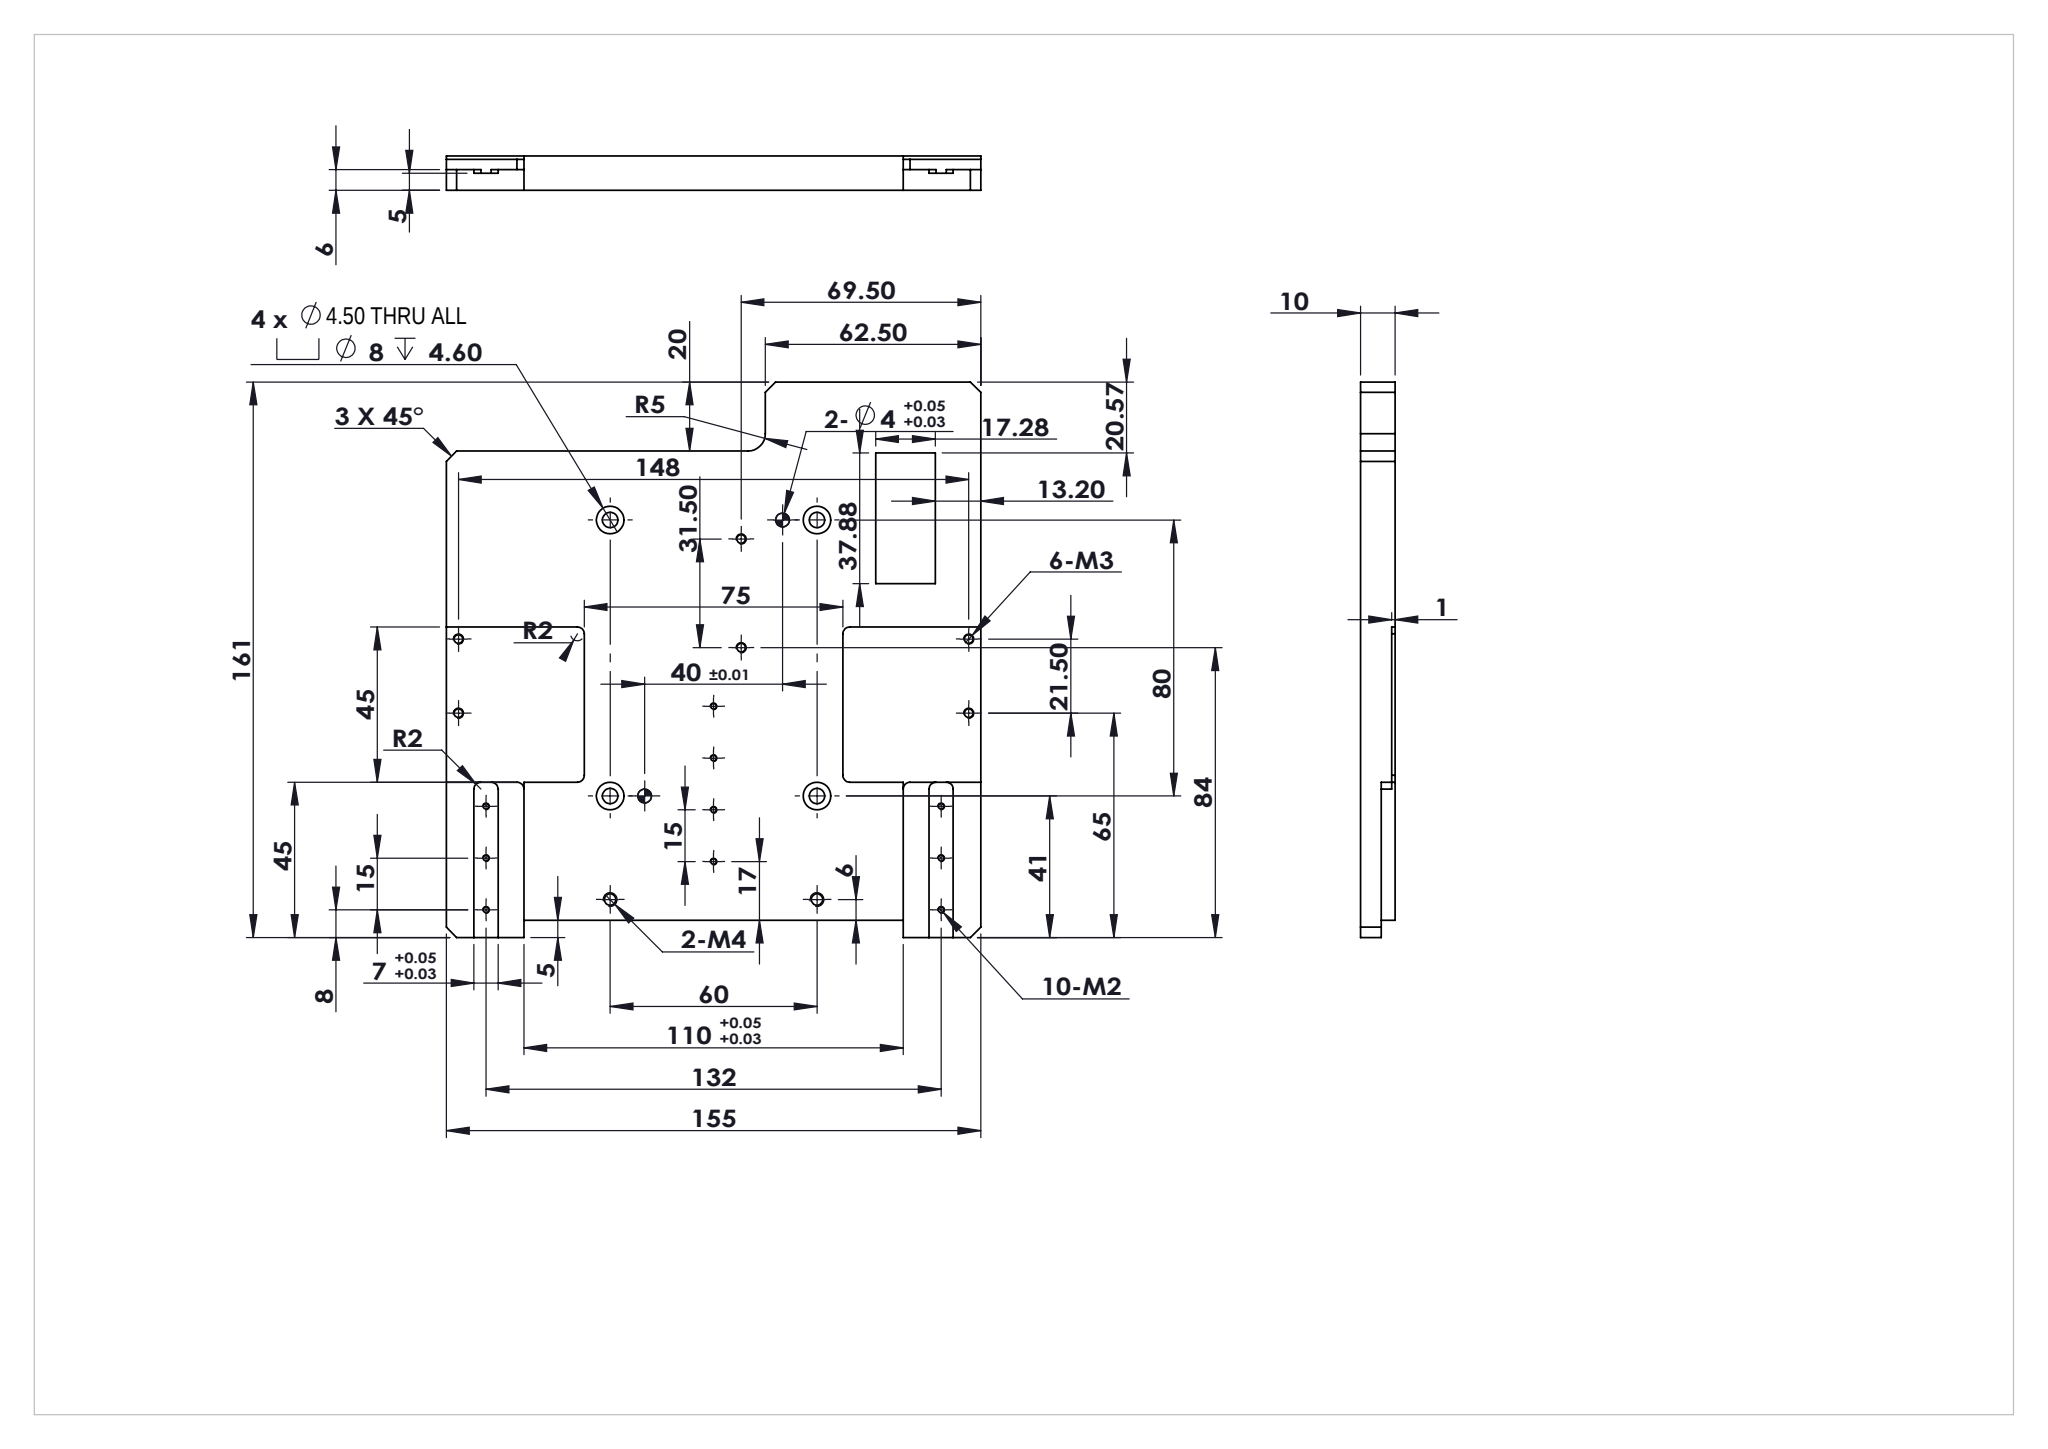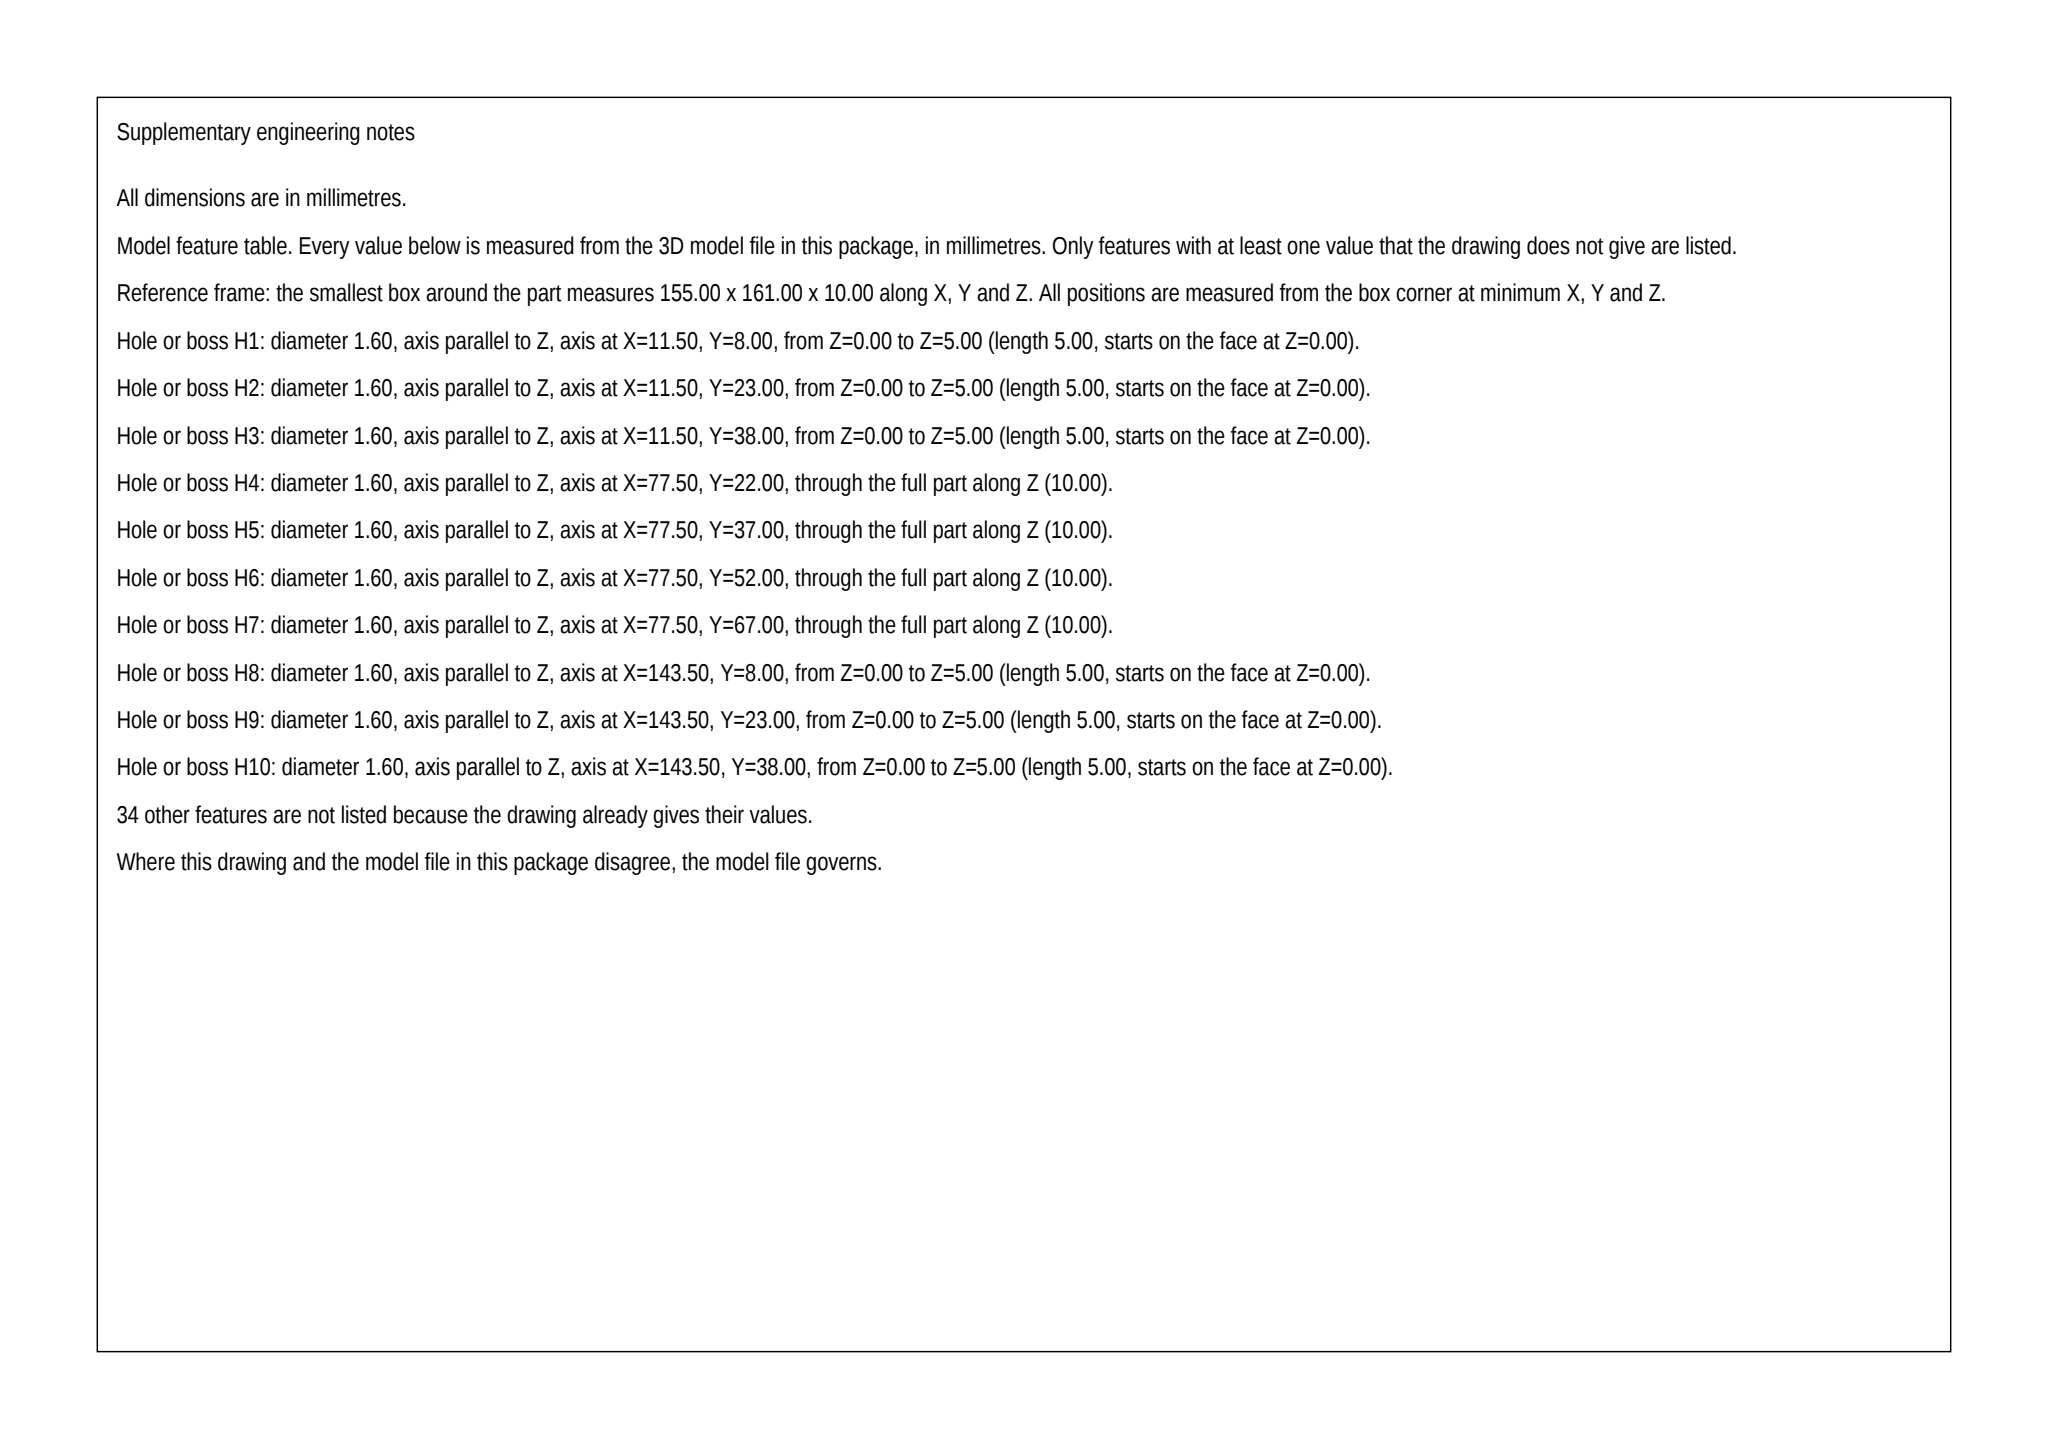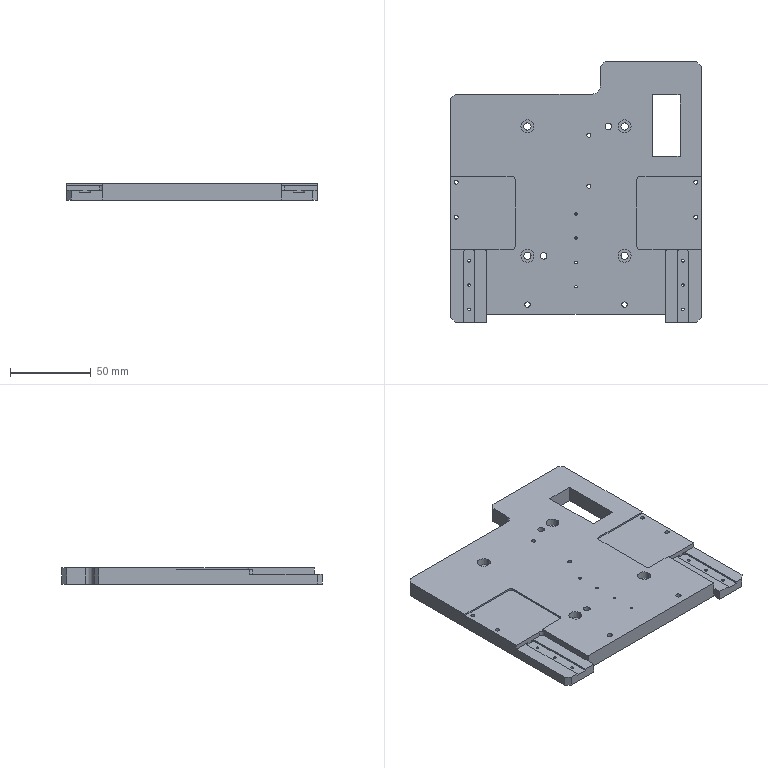Part | SolidWorks | mm | 1 solid | 114 faces | box 155 x 161 x 10 mm | volume 204444 mm3 | cylinder 67 | plane 47 | commonest cylinder face diameters 1.6 x20 4 x14 2.5 x12 8 x8 4.5 x8 3.3 x4 10 x1
build123d program:
from build123d import *

# Parameters (mm, degrees)
SKETCH1_2_W                                          = 155
SKETCH1_2_H                                          = 136
BOSS_EXTRUDE1_2_DEPTH                                = 10
SKETCH1_W                                            = 22.5
SKETCH1_H                                            = 5
BOSS_EXTRUDE1_DEPTH                                  = 10
SKETCH2_W                                            = 22.5
SKETCH2_H                                            = 45
CUT_EXTRUDE1_DEPTH                                   = 4
SKETCH4_W                                            = 62.5
SKETCH4_H                                            = 20
BOSS_EXTRUDE2_DEPTH                                  = 10
SKETCH5_W                                            = 7
SKETCH5_H                                            = 45
CUT_EXTRUDE2_DEPTH                                   = 1
FILLET1_2_R                                          = 2
SKETCH2_2_W                                          = 40
SKETCH2_2_H                                          = 45
CUT_EXTRUDE1_2_DEPTH                                 = 1
HOLE_SIZE_ACCORDING_TO_THE_TYPE_1_OF_HEX_D           = 4.5
HOLE_SIZE_ACCORDING_TO_THE_TYPE_1_OF_HEX_CBORE_D     = 8
HOLE_SIZE_ACCORDING_TO_THE_TYPE_1_OF_HEX_CBORE_DEPTH = 4.6
LPATTERN1_COUNT                                      = 2
LPATTERN1_PITCH                                      = 80
FILLET3_R                                            = 2
SKETCH5_2_R                                          = 2
CUT_EXTRUDE2_2_DEPTH                                 = 118.687
M3_TAPPED_HOLE1_D                                    = 2.5
FILLET4_R                                            = 5
M3_TAPPED_HOLE2_D                                    = 2.5
M2_TAPPED_HOLE1_D                                    = 1.6
FILLET1_R                                            = 2
M2_TAPPED_HOLE2_D                                    = 1.6
M4_TAPPED_HOLE1_D                                    = 3.3
CHAMFER1_SIZE                                        = 3
SKETCH16_W                                           = 17.28
SKETCH16_H                                           = 37.883
CUT_EXTRUDE3_DEPTH                                   = 45


with BuildPart() as part:
    # Sketch1_2 → Boss-Extrude1_2 (new body)
    with BuildSketch(Plane.XY):
        Rectangle(SKETCH1_2_W, SKETCH1_2_H)
    extrude(amount=BOSS_EXTRUDE1_2_DEPTH)

    # Sketch1 → Boss-Extrude1 (add)
    with BuildSketch(Plane.XY.offset(10)):
        with Locations((-66.25, -70.5)):
            Rectangle(SKETCH1_W, SKETCH1_H)
        with Locations((66.25, -70.5)):
            Rectangle(SKETCH1_W, SKETCH1_H)
    extrude(amount=-BOSS_EXTRUDE1_DEPTH)

    # Sketch2 → Cut-Extrude1 (cut)
    with BuildSketch(Plane.XY.offset(10)):
        with Locations((-66.25, -50.5)):
            Rectangle(SKETCH2_W, SKETCH2_H)
        with Locations((66.25, -50.5)):
            Rectangle(SKETCH2_W, SKETCH2_H)
    extrude(amount=-CUT_EXTRUDE1_DEPTH, mode=Mode.SUBTRACT)

    # Sketch4 → Boss-Extrude2 (add)
    with BuildSketch(Plane.XY.offset(10)):
        with Locations((46.25, 78)):
            Rectangle(SKETCH4_W, SKETCH4_H)
    extrude(amount=-BOSS_EXTRUDE2_DEPTH)

    # Sketch5 → Cut-Extrude2 (cut)
    with BuildSketch(Plane.XY.offset(6)):
        with Locations((-66, -50.5)):
            Rectangle(SKETCH5_W, SKETCH5_H)
        with Locations((66, -50.5)):
            Rectangle(SKETCH5_W, SKETCH5_H)
    extrude(amount=-CUT_EXTRUDE2_DEPTH, mode=Mode.SUBTRACT)

    # Fillet1_2
    fillet1_2_edges = [part.edges().sort_by_distance(p)[0] for p in [
        (62.5, -28, 5.5),
        (69.5, -28, 5.5),
        (-62.5, -28, 5.5),
        (-69.5, -28, 5.5),
    ]]
    fillet(fillet1_2_edges, radius=FILLET1_2_R)

    # Sketch2_2 → Cut-Extrude1_2 (cut)
    with BuildSketch(Plane.XY.offset(10)):
        with Locations((-57.5, -5.5)):
            Rectangle(SKETCH2_2_W, SKETCH2_2_H)
        with Locations((57.5, -5.5)):
            Rectangle(SKETCH2_2_W, SKETCH2_2_H)
    extrude(amount=-CUT_EXTRUDE1_2_DEPTH, mode=Mode.SUBTRACT)

    # Hole Size according to the type 1 of hex (through all)
    with Locations(Plane.XY.offset(10)):
        with Locations((-30, 48), (30, 48)):
            hole_size_according_to_the_type_1_of_hex = CounterBoreHole(HOLE_SIZE_ACCORDING_TO_THE_TYPE_1_OF_HEX_D / 2, HOLE_SIZE_ACCORDING_TO_THE_TYPE_1_OF_HEX_CBORE_D / 2, HOLE_SIZE_ACCORDING_TO_THE_TYPE_1_OF_HEX_CBORE_DEPTH)

    # LPattern1: Hole Size according to the type 1 of hex ×2
    with Locations(*[(0, -i * LPATTERN1_PITCH, 0) for i in range(1, LPATTERN1_COUNT)]):
        add(hole_size_according_to_the_type_1_of_hex, mode=Mode.SUBTRACT)

    # Fillet3
    fillet3_edges = [part.edges().sort_by_distance(p)[0] for p in [
        (-55, -28, 7.5),
        (55, -28, 7.5),
    ]]
    fillet(fillet3_edges, radius=FILLET3_R)

    # Sketch5_2 → Cut-Extrude2_2 (cut, through all)
    with BuildSketch(Plane.XY.offset(10)):
        with Locations((20, 48)):
            Circle(SKETCH5_2_R)
        with Locations((-20, -32)):
            Circle(SKETCH5_2_R)
    extrude(amount=-CUT_EXTRUDE2_2_DEPTH, mode=Mode.SUBTRACT)

    # M3 Tapped Hole1 (through all)
    with Locations(Plane.XY.offset(10)):
        with Locations((8, 42.5), (8, 11)):
            Hole(M3_TAPPED_HOLE1_D / 2)

    # Fillet4
    fillet4_edges = [part.edges().sort_by_distance(p)[0] for p in [
        (15, 68, 5),
    ]]
    fillet(fillet4_edges, radius=FILLET4_R)

    # M3 Tapped Hole2 (through all)
    with Locations(Plane.XY.offset(9)):
        with Locations((-74, 13.5), (-74, -8), (74, -8), (74, 13.5)):
            Hole(M3_TAPPED_HOLE2_D / 2)

    # M2 Tapped Hole1 (through all)
    with Locations(Plane.XY.offset(5)):
        with Locations((-66, -35), (-66, -50), (-66, -65), (66, -65), (66, -50), (66, -35)):
            Hole(M2_TAPPED_HOLE1_D / 2)

    # Fillet1
    fillet1_edges = [part.edges().sort_by_distance(p)[0] for p in [
        (-37.5, -28, 9.5),
        (-37.5, 17, 9.5),
        (37.5, -28, 9.5),
        (37.5, 17, 9.5),
    ]]
    fillet(fillet1_edges, radius=FILLET1_R)

    # M2 Tapped Hole2 (through all)
    with Locations(Plane.XY.offset(10)):
        with Locations((0, -6), (0, -21), (0, -36), (0, -51)):
            Hole(M2_TAPPED_HOLE2_D / 2)

    # M4 Tapped Hole1 (through all)
    with Locations(Plane.XY.offset(10)):
        with Locations((-30, -62), (30, -62)):
            Hole(M4_TAPPED_HOLE1_D / 2)

    # Chamfer1
    chamfer1_edges = [part.edges().sort_by_distance(p)[0] for p in [
        (77.5, 88, 5),
        (15, 88, 5),
        (-77.5, 68, 5),
        (77.5, -73, 3),
        (-77.5, -73, 3),
    ]]
    chamfer(chamfer1_edges, length=CHAMFER1_SIZE)

    # Sketch16 → Cut-Extrude3 (cut)
    with BuildSketch(Plane.XY.offset(10)):
        with Locations((55.661, 48.492)):
            Rectangle(SKETCH16_W, SKETCH16_H)
    extrude(amount=-CUT_EXTRUDE3_DEPTH, mode=Mode.SUBTRACT)


solid = part.part